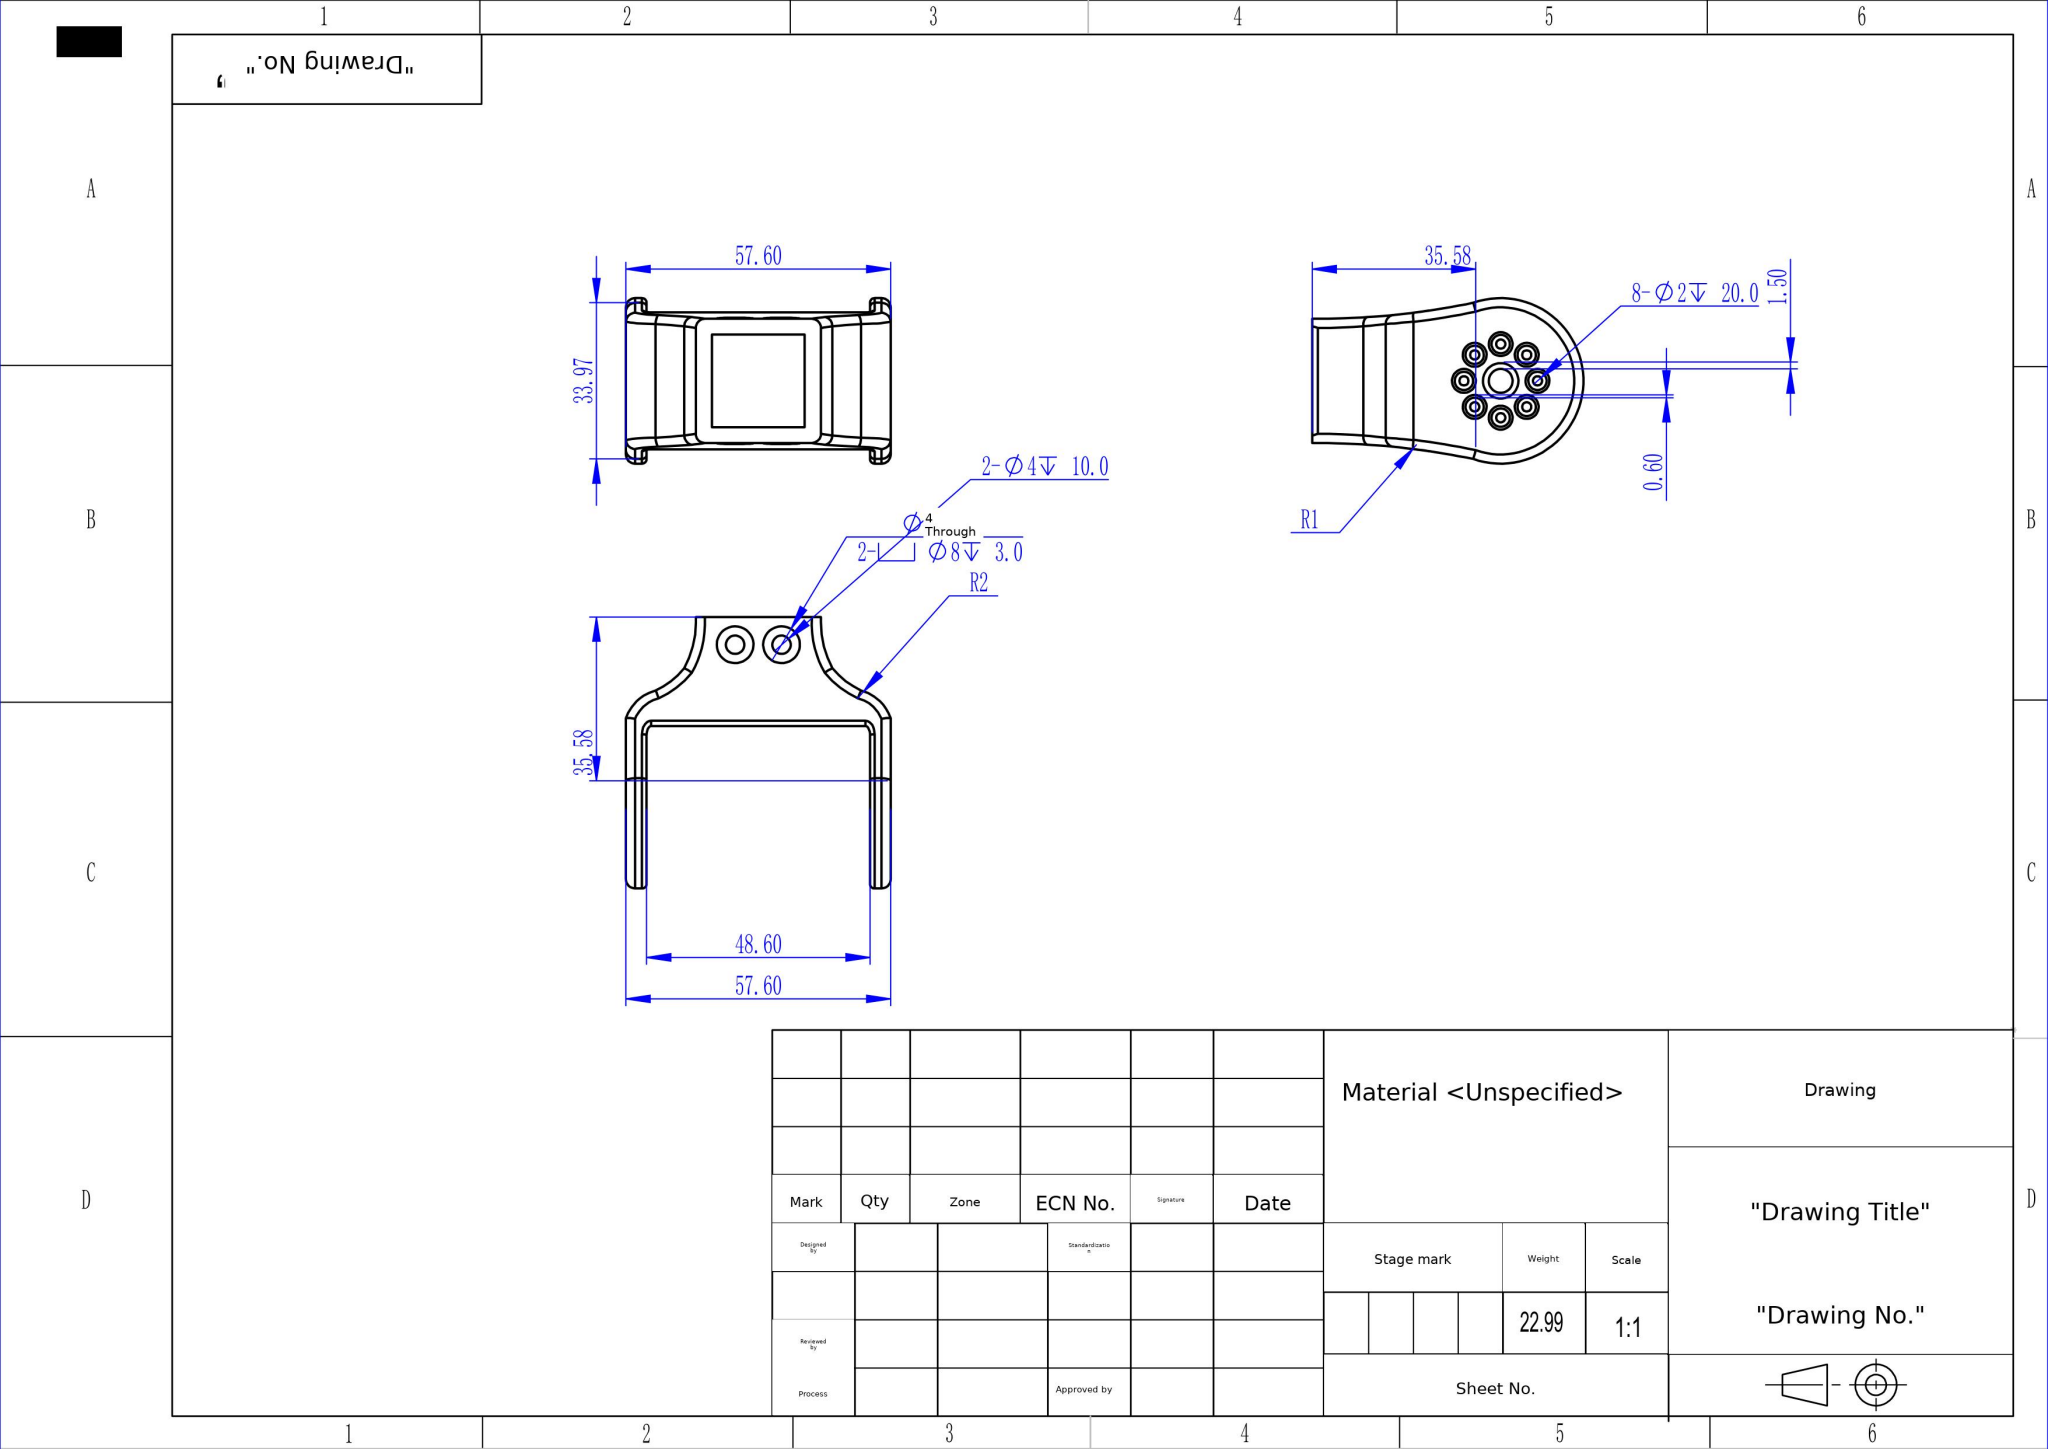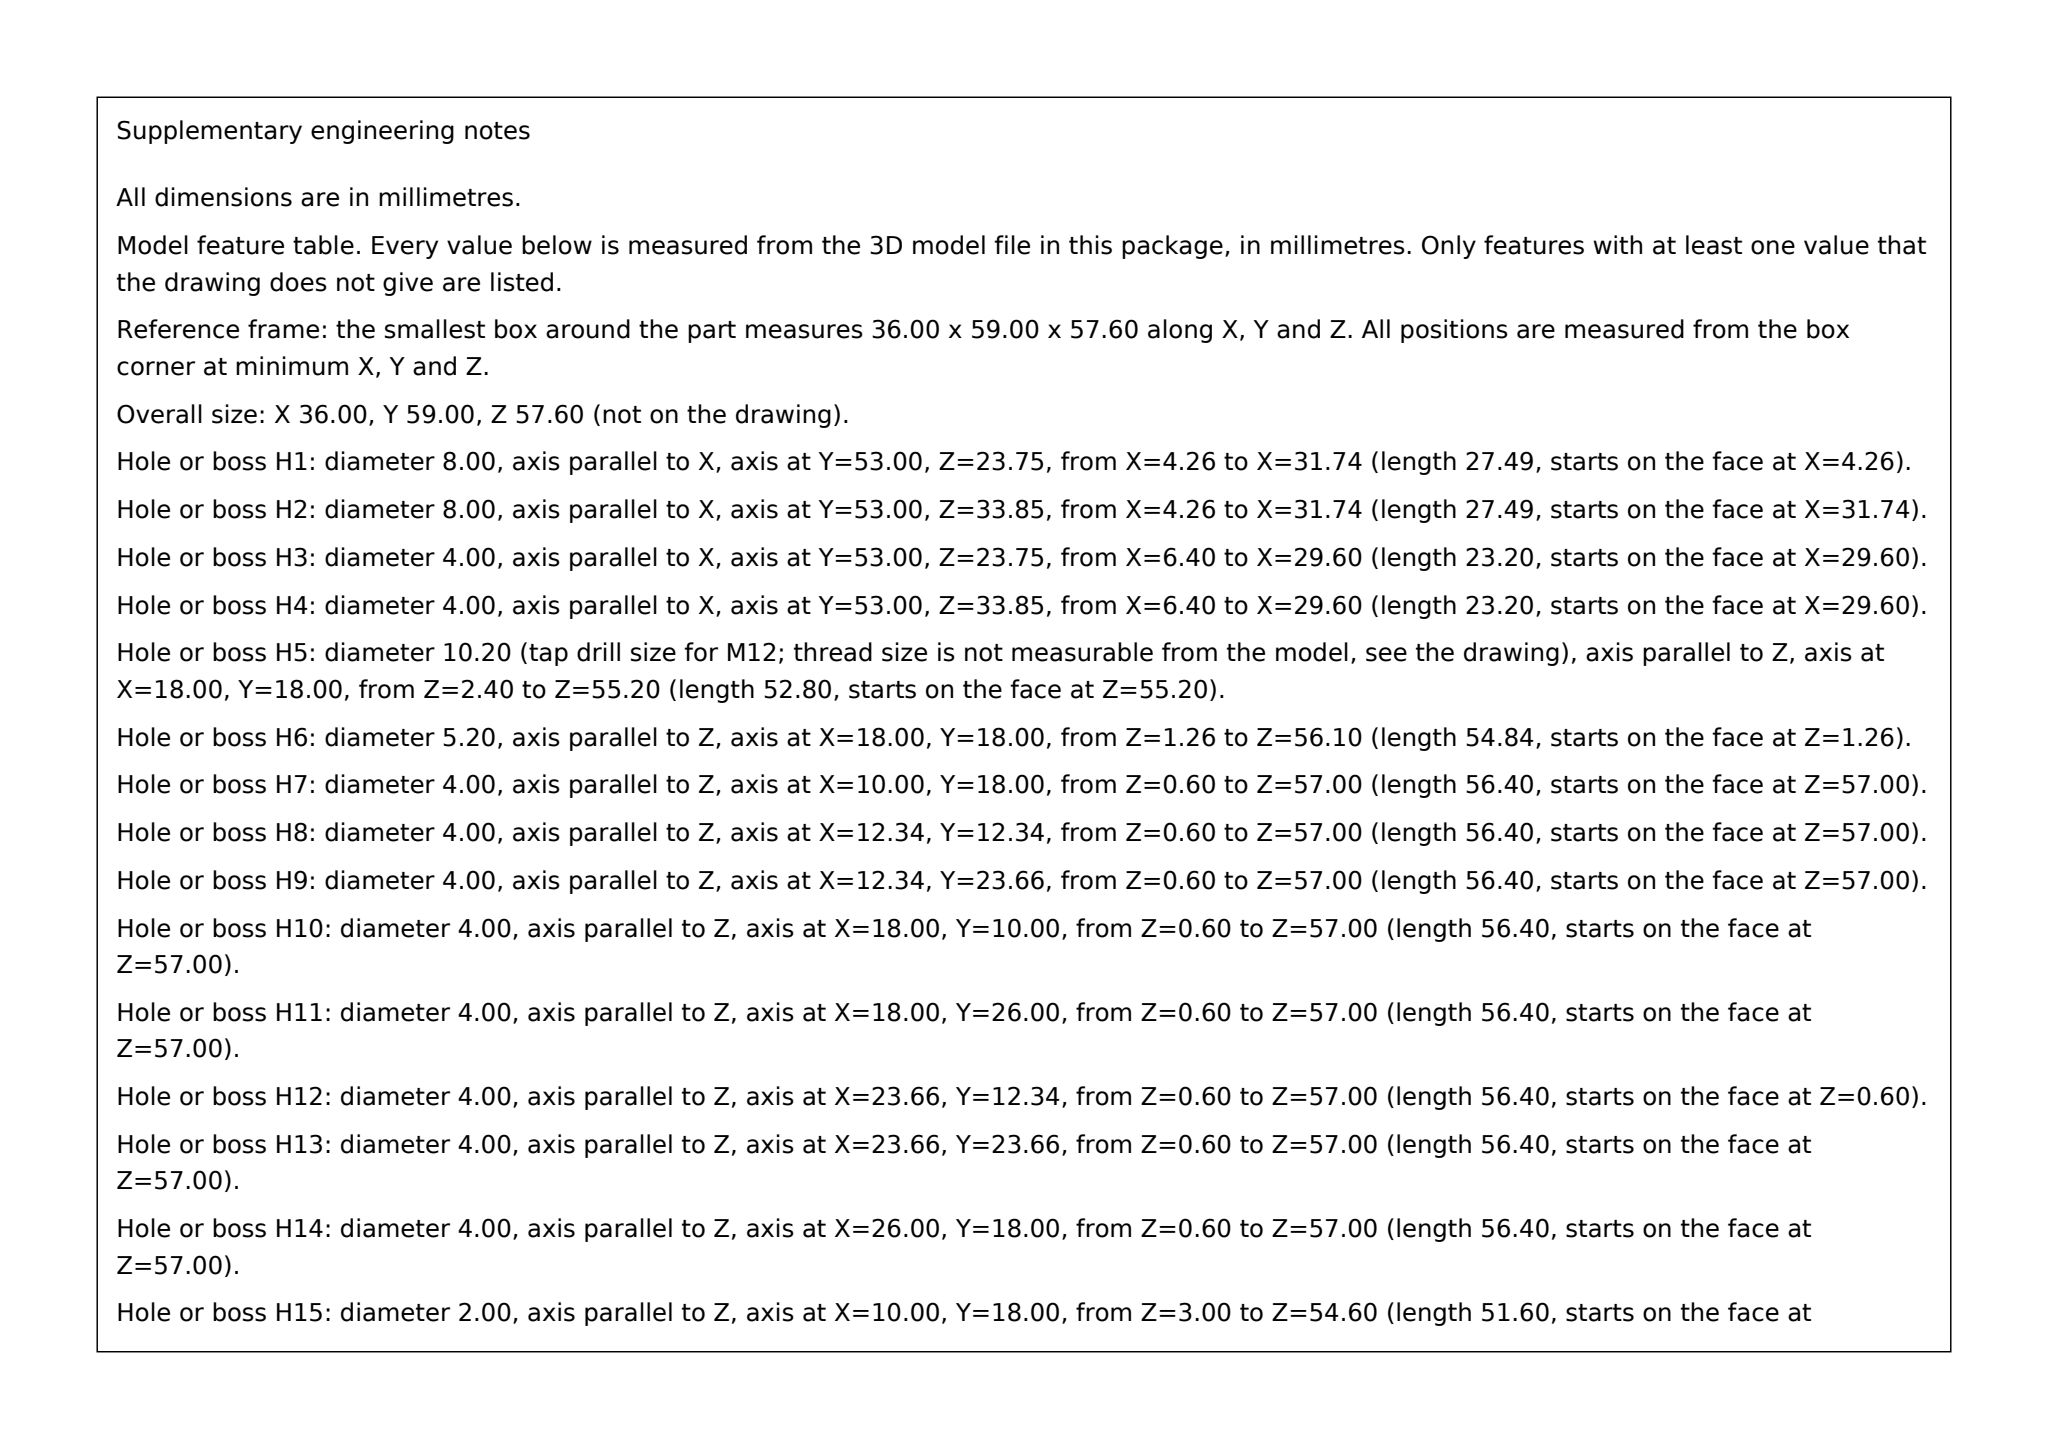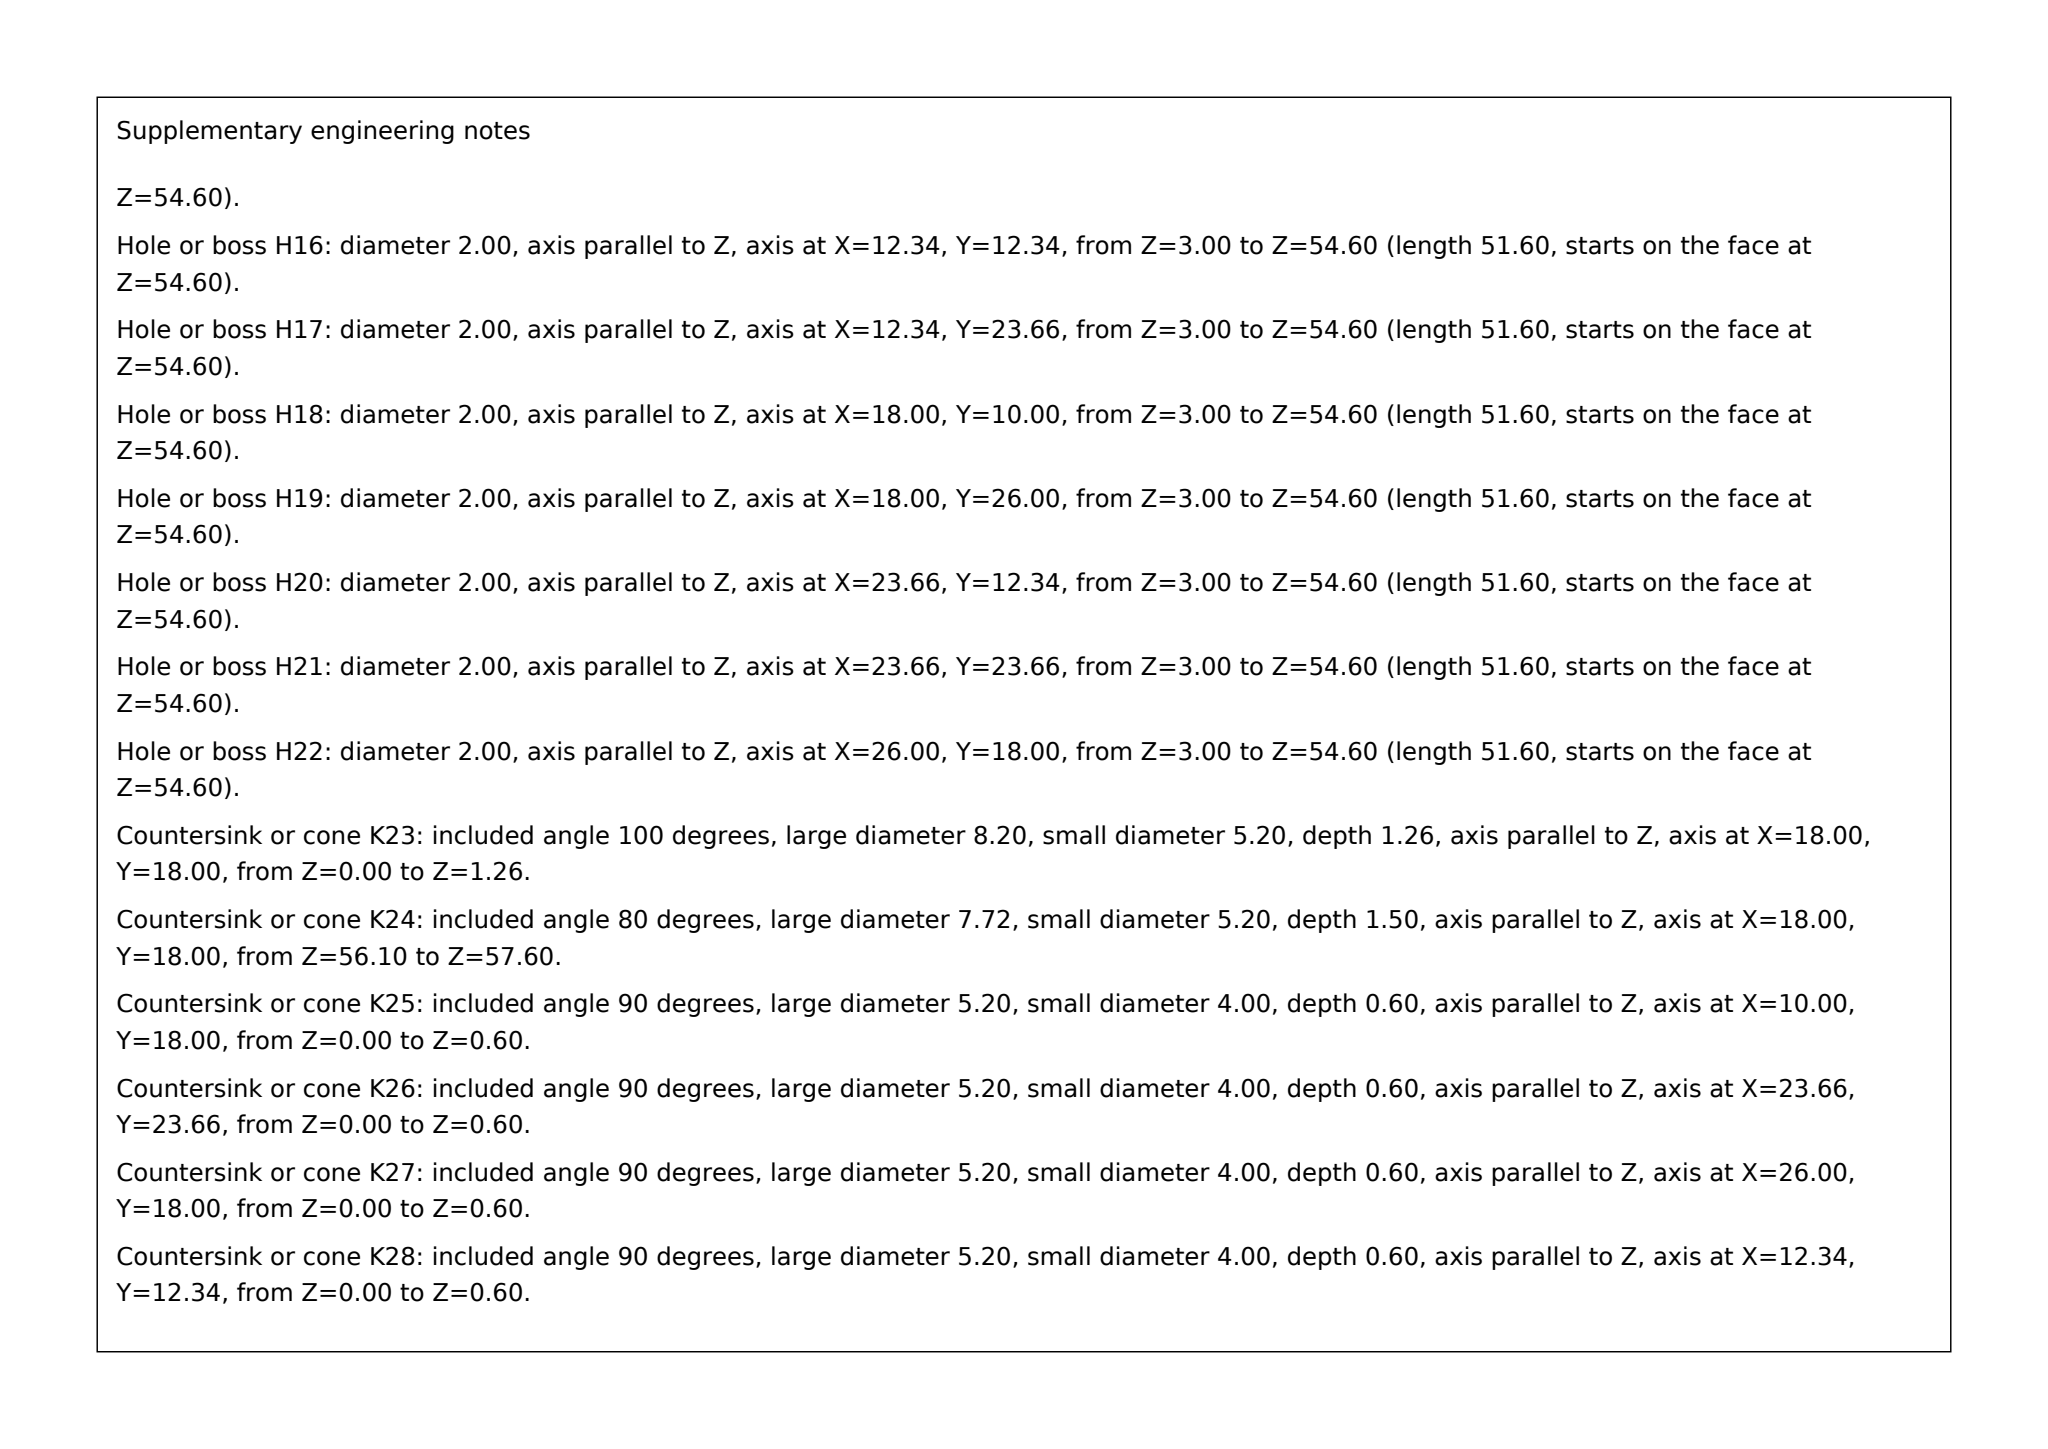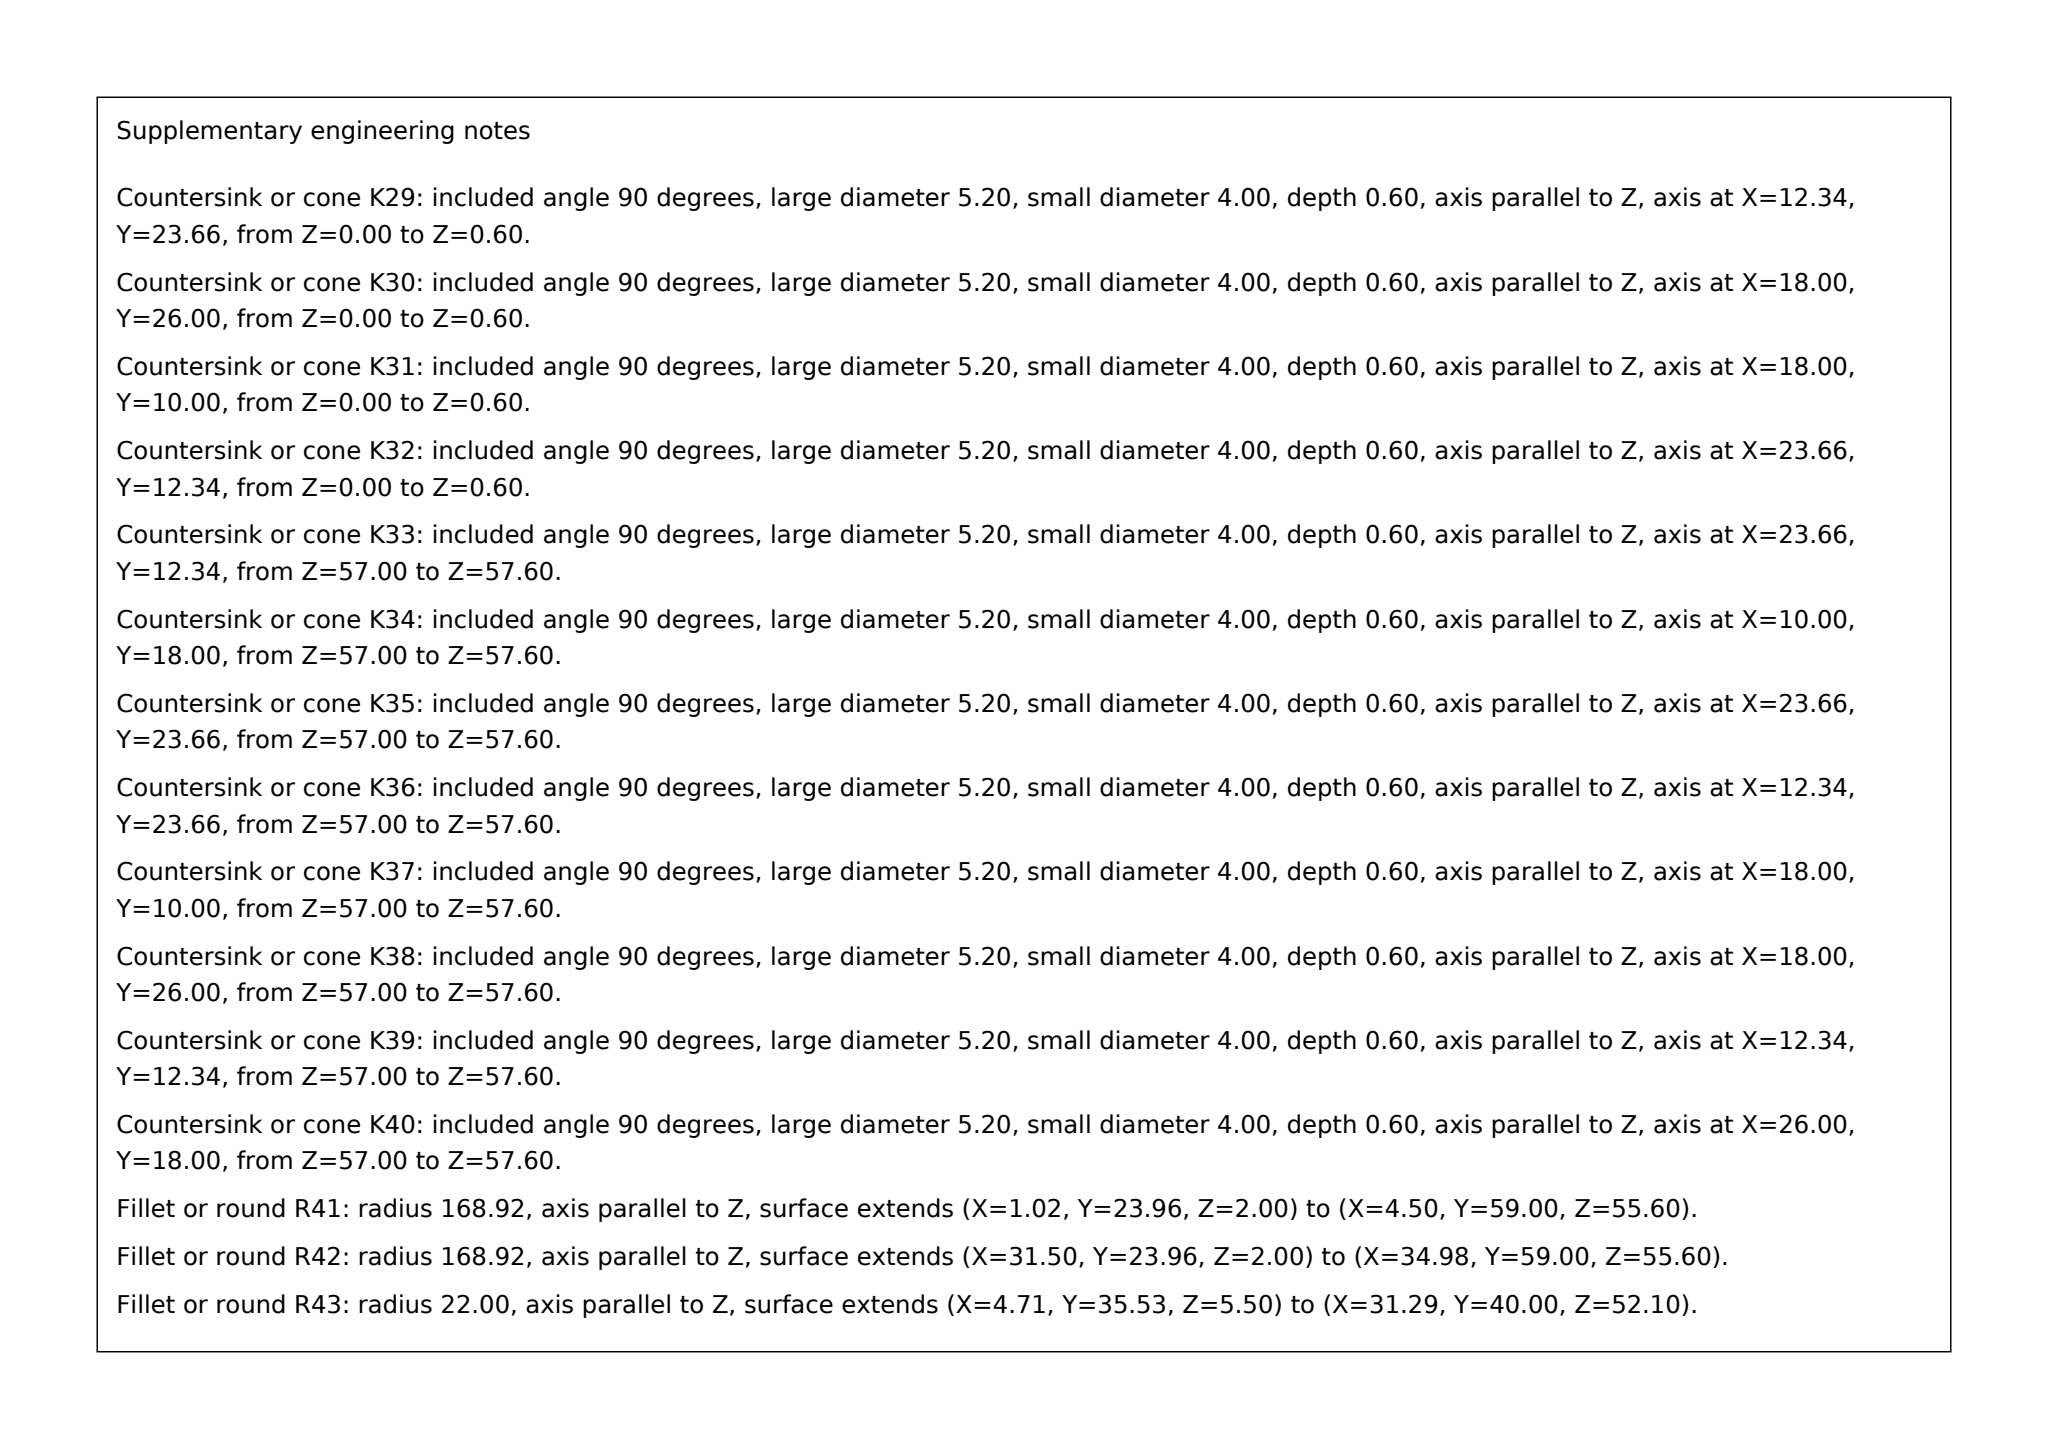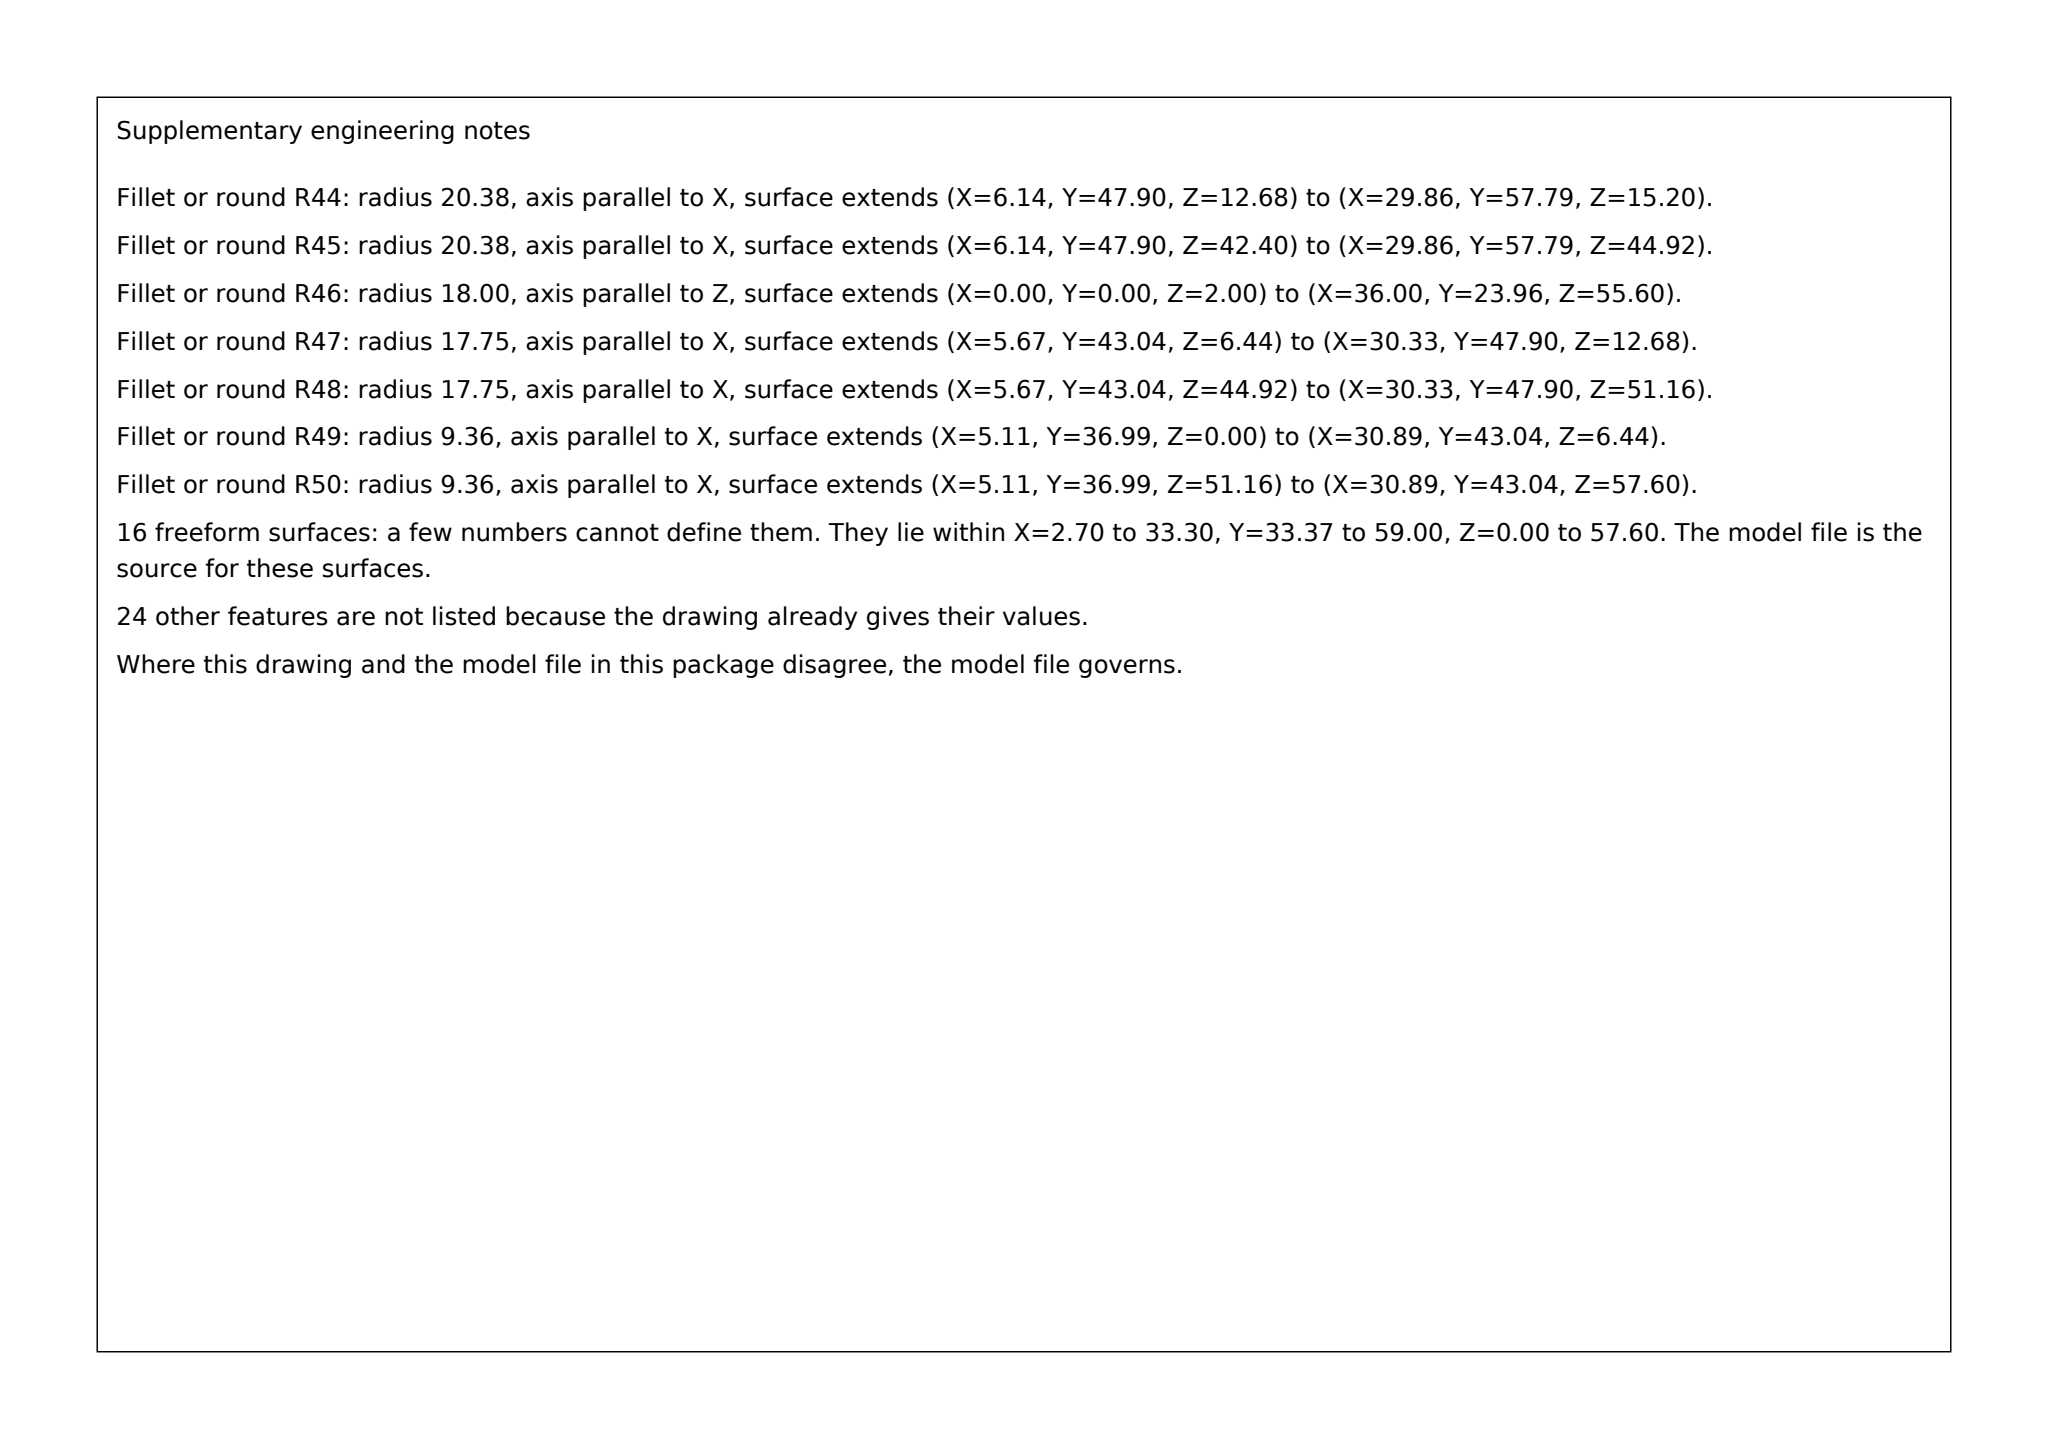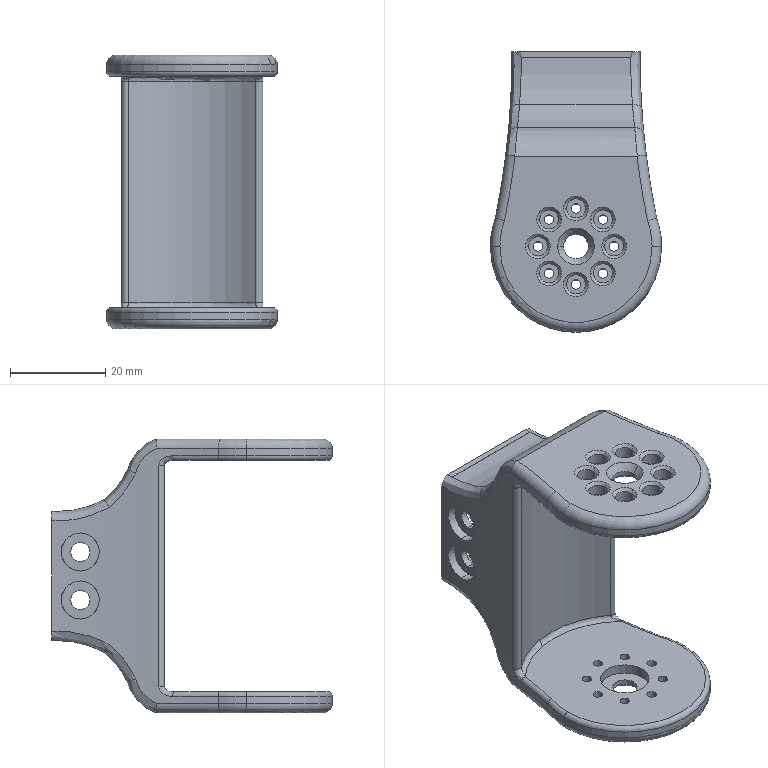Part | SolidWorks | mm | 1 solid | 216 faces | box 36 x 59 x 57.6 mm | volume 22990 mm3 | cylinder 108 | cone 36 | plane 34 | torus 22 | spline 16 | commonest cylinder face diameters 4 x40 2 x35 8 x8 36 x6 5.2 x4 10.2 x4 40.754 x3 337.835 x3